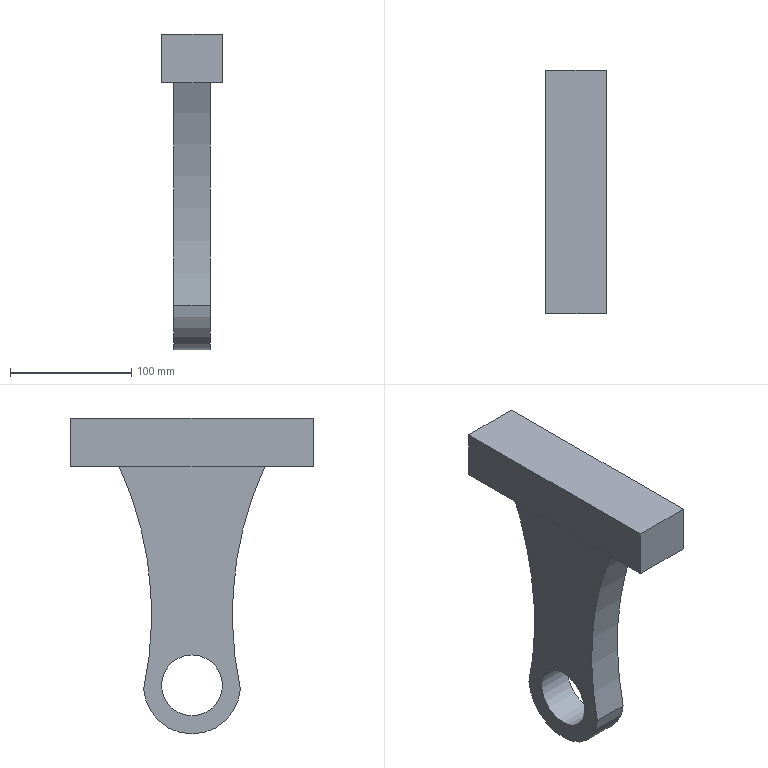Component | NX | HAMMER_HEAD_3 | 1 solid | 12 faces | box 50 x 200 x 260 mm | volume 846348 mm3 | plane 8 | cylinder 4 | commonest cylinder face diameters 580.798 x2 80 x1 50 x1
STEP:
#1=CARTESIAN_POINT('',(0.,0.,0.));
#2=DIRECTION('',(0.,0.,1.));
#3=DIRECTION('',(1.,0.,0.));
#4=AXIS2_PLACEMENT_3D('',#1,#2,#3);
#5=CARTESIAN_POINT('',(660.371,-609.017,1839.037));
#6=VERTEX_POINT('',#5);
#7=CARTESIAN_POINT('',(660.371,-688.747,1839.037));
#8=VERTEX_POINT('',#7);
#9=CARTESIAN_POINT('',(660.371,-648.882,1842.318));
#10=DIRECTION('',(-1.,0.,0.));
#11=DIRECTION('',(0.,0.,1.));
#12=AXIS2_PLACEMENT_3D('',#9,#10,#11);
#13=CIRCLE('',#12,40.);
#14=CARTESIAN_POINT('',(630.371,-648.882,1842.318));
#15=DIRECTION('',(1.,0.,0.));
#16=DIRECTION('',(0.,0.,-1.));
#17=AXIS2_PLACEMENT_3D('',#14,#15,#16);
#18=CYLINDRICAL_SURFACE('',#17,40.);
#19=CARTESIAN_POINT('',(3.142,30.));
#20=DIRECTION('',(-1.,0.));
#21=VECTOR('',#20,1.);
#22=LINE('',#19,#21);
#23=(GEOMETRIC_REPRESENTATION_CONTEXT(2)PARAMETRIC_REPRESENTATION_CONTEXT()REPRESENTATION_CONTEXT('',''));
#24=DEFINITIONAL_REPRESENTATION('',(#22),#23);
#25=PCURVE('',#18,#24);
#26=CARTESIAN_POINT('',(660.371,-648.882,1842.318));
#27=DIRECTION('',(-1.,0.,0.));
#28=DIRECTION('',(0.,0.,1.));
#29=AXIS2_PLACEMENT_3D('',#26,#27,#28);
#30=PLANE('',#29);
#31=CARTESIAN_POINT('',(0.,0.));
#32=DIRECTION('',(1.,0.));
#33=AXIS2_PLACEMENT_2D('',#31,#32);
#34=CIRCLE('',#33,40.);
#35=(GEOMETRIC_REPRESENTATION_CONTEXT(2)PARAMETRIC_REPRESENTATION_CONTEXT()REPRESENTATION_CONTEXT('',''));
#36=DEFINITIONAL_REPRESENTATION('',(#34),#35);
#37=PCURVE('',#30,#36);
#38=SURFACE_CURVE('',#13,(#25,#37),.PCURVE_S1.);
#39=EDGE_CURVE('',#6,#8,#38,.T.);
#40=ORIENTED_EDGE('',*,*,#39,.T.);
#41=CARTESIAN_POINT('',(630.371,-688.747,1839.037));
#42=VERTEX_POINT('',#41);
#43=CARTESIAN_POINT('',(630.371,-688.747,1839.037));
#44=DIRECTION('',(1.,0.,0.));
#45=VECTOR('',#44,1.);
#46=LINE('',#43,#45);
#47=CARTESIAN_POINT('',(-1.489,0.));
#48=DIRECTION('',(0.,1.));
#49=VECTOR('',#48,1.);
#50=LINE('',#47,#49);
#51=(GEOMETRIC_REPRESENTATION_CONTEXT(2)PARAMETRIC_REPRESENTATION_CONTEXT()REPRESENTATION_CONTEXT('',''));
#52=DEFINITIONAL_REPRESENTATION('',(#50),#51);
#53=PCURVE('',#18,#52);
#54=CARTESIAN_POINT('',(630.371,-972.544,1900.606));
#55=DIRECTION('',(1.,0.,0.));
#56=DIRECTION('',(0.,0.,-1.));
#57=AXIS2_PLACEMENT_3D('',#54,#55,#56);
#58=CYLINDRICAL_SURFACE('',#57,290.399);
#59=CARTESIAN_POINT('',(1.357,0.));
#60=DIRECTION('',(0.,1.));
#61=VECTOR('',#60,1.);
#62=LINE('',#59,#61);
#63=(GEOMETRIC_REPRESENTATION_CONTEXT(2)PARAMETRIC_REPRESENTATION_CONTEXT()REPRESENTATION_CONTEXT('',''));
#64=DEFINITIONAL_REPRESENTATION('',(#62),#63);
#65=PCURVE('',#58,#64);
#66=SURFACE_CURVE('',#46,(#53,#65),.PCURVE_S1.);
#67=EDGE_CURVE('',#42,#8,#66,.T.);
#68=ORIENTED_EDGE('',*,*,#67,.F.);
#69=CARTESIAN_POINT('',(630.371,-609.017,1839.037));
#70=VERTEX_POINT('',#69);
#71=CARTESIAN_POINT('',(630.371,-648.882,1842.318));
#72=DIRECTION('',(-1.,0.,0.));
#73=DIRECTION('',(0.,0.,1.));
#74=AXIS2_PLACEMENT_3D('',#71,#72,#73);
#75=CIRCLE('',#74,40.);
#76=CARTESIAN_POINT('',(3.142,0.));
#77=DIRECTION('',(-1.,0.));
#78=VECTOR('',#77,1.);
#79=LINE('',#76,#78);
#80=(GEOMETRIC_REPRESENTATION_CONTEXT(2)PARAMETRIC_REPRESENTATION_CONTEXT()REPRESENTATION_CONTEXT('',''));
#81=DEFINITIONAL_REPRESENTATION('',(#79),#80);
#82=PCURVE('',#18,#81);
#83=CARTESIAN_POINT('',(630.371,-648.882,1842.318));
#84=DIRECTION('',(-1.,0.,0.));
#85=DIRECTION('',(0.,0.,1.));
#86=AXIS2_PLACEMENT_3D('',#83,#84,#85);
#87=PLANE('',#86);
#88=CARTESIAN_POINT('',(0.,0.));
#89=DIRECTION('',(1.,0.));
#90=AXIS2_PLACEMENT_2D('',#88,#89);
#91=CIRCLE('',#90,40.);
#92=(GEOMETRIC_REPRESENTATION_CONTEXT(2)PARAMETRIC_REPRESENTATION_CONTEXT()REPRESENTATION_CONTEXT('',''));
#93=DEFINITIONAL_REPRESENTATION('',(#91),#92);
#94=PCURVE('',#87,#93);
#95=SURFACE_CURVE('',#75,(#82,#94),.PCURVE_S1.);
#96=EDGE_CURVE('',#70,#42,#95,.T.);
#97=ORIENTED_EDGE('',*,*,#96,.F.);
#98=CARTESIAN_POINT('',(630.371,-609.017,1839.037));
#99=DIRECTION('',(1.,0.,0.));
#100=VECTOR('',#99,1.);
#101=LINE('',#98,#100);
#102=CARTESIAN_POINT('',(1.489,0.));
#103=DIRECTION('',(0.,1.));
#104=VECTOR('',#103,1.);
#105=LINE('',#102,#104);
#106=(GEOMETRIC_REPRESENTATION_CONTEXT(2)PARAMETRIC_REPRESENTATION_CONTEXT()REPRESENTATION_CONTEXT('',''));
#107=DEFINITIONAL_REPRESENTATION('',(#105),#106);
#108=PCURVE('',#18,#107);
#109=CARTESIAN_POINT('',(630.371,-325.22,1900.606));
#110=DIRECTION('',(1.,0.,0.));
#111=DIRECTION('',(0.,0.,-1.));
#112=AXIS2_PLACEMENT_3D('',#109,#110,#111);
#113=CYLINDRICAL_SURFACE('',#112,290.399);
#114=CARTESIAN_POINT('',(4.926,0.));
#115=DIRECTION('',(0.,1.));
#116=VECTOR('',#115,1.);
#117=LINE('',#114,#116);
#118=(GEOMETRIC_REPRESENTATION_CONTEXT(2)PARAMETRIC_REPRESENTATION_CONTEXT()REPRESENTATION_CONTEXT('',''));
#119=DEFINITIONAL_REPRESENTATION('',(#117),#118);
#120=PCURVE('',#113,#119);
#121=SURFACE_CURVE('',#101,(#108,#120),.PCURVE_S1.);
#122=EDGE_CURVE('',#70,#6,#121,.T.);
#123=ORIENTED_EDGE('',*,*,#122,.T.);
#124=EDGE_LOOP('',(#40,#68,#97,#123));
#125=FACE_BOUND('',#124,.T.);
#126=ADVANCED_FACE('',(#125),#18,.T.);
#127=ORIENTED_EDGE('',*,*,#67,.F.);
#128=CARTESIAN_POINT('',(630.371,-708.882,2022.318));
#129=VERTEX_POINT('',#128);
#130=CARTESIAN_POINT('',(630.371,-972.544,1900.606));
#131=DIRECTION('',(1.,0.,0.));
#132=DIRECTION('',(0.,0.,1.));
#133=AXIS2_PLACEMENT_3D('',#130,#131,#132);
#134=CIRCLE('',#133,290.399);
#135=CARTESIAN_POINT('',(-3.142,0.));
#136=DIRECTION('',(1.,0.));
#137=VECTOR('',#136,1.);
#138=LINE('',#135,#137);
#139=(GEOMETRIC_REPRESENTATION_CONTEXT(2)PARAMETRIC_REPRESENTATION_CONTEXT()REPRESENTATION_CONTEXT('',''));
#140=DEFINITIONAL_REPRESENTATION('',(#138),#139);
#141=PCURVE('',#58,#140);
#142=CARTESIAN_POINT('',(348.687,-323.662));
#143=CARTESIAN_POINT('',(348.687,-826.648));
#144=CARTESIAN_POINT('',(-86.911,-575.155));
#145=CARTESIAN_POINT('',(-522.509,-323.662));
#146=CARTESIAN_POINT('',(-86.911,-72.169));
#147=CARTESIAN_POINT('',(348.687,179.323));
#148=CARTESIAN_POINT('',(348.687,-323.662));
#149=(BOUNDED_CURVE()B_SPLINE_CURVE(2,(#142,#143,#144,#145,#146,#147,#148),.UNSPECIFIED.,.T.,.F.)B_SPLINE_CURVE_WITH_KNOTS((1,2,2,2,2,1),(-2.094,0.,2.094,4.189,6.283,8.378),.UNSPECIFIED.)CURVE()GEOMETRIC_REPRESENTATION_ITEM()RATIONAL_B_SPLINE_CURVE((1.,0.5,1.,0.5,1.,0.5,1.))REPRESENTATION_ITEM(''));
#150=(GEOMETRIC_REPRESENTATION_CONTEXT(2)PARAMETRIC_REPRESENTATION_CONTEXT()REPRESENTATION_CONTEXT('',''));
#151=DEFINITIONAL_REPRESENTATION('',(#149),#150);
#152=PCURVE('',#87,#151);
#153=SURFACE_CURVE('',#134,(#141,#152),.PCURVE_S1.);
#154=EDGE_CURVE('',#42,#129,#153,.T.);
#155=ORIENTED_EDGE('',*,*,#154,.T.);
#156=CARTESIAN_POINT('',(660.371,-708.882,2022.318));
#157=VERTEX_POINT('',#156);
#158=CARTESIAN_POINT('',(630.371,-708.882,2022.318));
#159=DIRECTION('',(1.,0.,0.));
#160=VECTOR('',#159,1.);
#161=LINE('',#158,#160);
#162=CARTESIAN_POINT('',(2.003,0.));
#163=DIRECTION('',(0.,1.));
#164=VECTOR('',#163,1.);
#165=LINE('',#162,#164);
#166=(GEOMETRIC_REPRESENTATION_CONTEXT(2)PARAMETRIC_REPRESENTATION_CONTEXT()REPRESENTATION_CONTEXT('',''));
#167=DEFINITIONAL_REPRESENTATION('',(#165),#166);
#168=PCURVE('',#58,#167);
#169=CARTESIAN_POINT('',(660.371,-648.882,2022.318));
#170=DIRECTION('',(0.,-0.,1.));
#171=DIRECTION('',(0.,1.,0.));
#172=AXIS2_PLACEMENT_3D('',#169,#170,#171);
#173=PLANE('',#172);
#174=CARTESIAN_POINT('',(-60.,30.));
#175=DIRECTION('',(0.,-1.));
#176=VECTOR('',#175,1.);
#177=LINE('',#174,#176);
#178=(GEOMETRIC_REPRESENTATION_CONTEXT(2)PARAMETRIC_REPRESENTATION_CONTEXT()REPRESENTATION_CONTEXT('',''));
#179=DEFINITIONAL_REPRESENTATION('',(#177),#178);
#180=PCURVE('',#173,#179);
#181=SURFACE_CURVE('',#161,(#168,#180),.PCURVE_S1.);
#182=EDGE_CURVE('',#129,#157,#181,.T.);
#183=ORIENTED_EDGE('',*,*,#182,.T.);
#184=CARTESIAN_POINT('',(660.371,-972.544,1900.606));
#185=DIRECTION('',(1.,0.,0.));
#186=DIRECTION('',(0.,0.,1.));
#187=AXIS2_PLACEMENT_3D('',#184,#185,#186);
#188=CIRCLE('',#187,290.399);
#189=CARTESIAN_POINT('',(-3.142,30.));
#190=DIRECTION('',(1.,0.));
#191=VECTOR('',#190,1.);
#192=LINE('',#189,#191);
#193=(GEOMETRIC_REPRESENTATION_CONTEXT(2)PARAMETRIC_REPRESENTATION_CONTEXT()REPRESENTATION_CONTEXT('',''));
#194=DEFINITIONAL_REPRESENTATION('',(#192),#193);
#195=PCURVE('',#58,#194);
#196=CARTESIAN_POINT('',(348.687,-323.662));
#197=CARTESIAN_POINT('',(348.687,-826.648));
#198=CARTESIAN_POINT('',(-86.911,-575.155));
#199=CARTESIAN_POINT('',(-522.509,-323.662));
#200=CARTESIAN_POINT('',(-86.911,-72.169));
#201=CARTESIAN_POINT('',(348.687,179.323));
#202=CARTESIAN_POINT('',(348.687,-323.662));
#203=(BOUNDED_CURVE()B_SPLINE_CURVE(2,(#196,#197,#198,#199,#200,#201,#202),.UNSPECIFIED.,.T.,.F.)B_SPLINE_CURVE_WITH_KNOTS((1,2,2,2,2,1),(-2.094,0.,2.094,4.189,6.283,8.378),.UNSPECIFIED.)CURVE()GEOMETRIC_REPRESENTATION_ITEM()RATIONAL_B_SPLINE_CURVE((1.,0.5,1.,0.5,1.,0.5,1.))REPRESENTATION_ITEM(''));
#204=(GEOMETRIC_REPRESENTATION_CONTEXT(2)PARAMETRIC_REPRESENTATION_CONTEXT()REPRESENTATION_CONTEXT('',''));
#205=DEFINITIONAL_REPRESENTATION('',(#203),#204);
#206=PCURVE('',#30,#205);
#207=SURFACE_CURVE('',#188,(#195,#206),.PCURVE_S1.);
#208=EDGE_CURVE('',#8,#157,#207,.T.);
#209=ORIENTED_EDGE('',*,*,#208,.F.);
#210=EDGE_LOOP('',(#127,#155,#183,#209));
#211=FACE_BOUND('',#210,.F.);
#212=ADVANCED_FACE('',(#211),#58,.F.);
#213=CARTESIAN_POINT('',(630.371,-588.882,2022.318));
#214=VERTEX_POINT('',#213);
#215=CARTESIAN_POINT('',(660.371,-588.882,2022.318));
#216=VERTEX_POINT('',#215);
#217=CARTESIAN_POINT('',(630.371,-588.882,2022.318));
#218=DIRECTION('',(1.,0.,0.));
#219=VECTOR('',#218,1.);
#220=LINE('',#217,#219);
#221=CARTESIAN_POINT('',(4.28,0.));
#222=DIRECTION('',(0.,1.));
#223=VECTOR('',#222,1.);
#224=LINE('',#221,#223);
#225=(GEOMETRIC_REPRESENTATION_CONTEXT(2)PARAMETRIC_REPRESENTATION_CONTEXT()REPRESENTATION_CONTEXT('',''));
#226=DEFINITIONAL_REPRESENTATION('',(#224),#225);
#227=PCURVE('',#113,#226);
#228=CARTESIAN_POINT('',(60.,30.));
#229=DIRECTION('',(0.,-1.));
#230=VECTOR('',#229,1.);
#231=LINE('',#228,#230);
#232=(GEOMETRIC_REPRESENTATION_CONTEXT(2)PARAMETRIC_REPRESENTATION_CONTEXT()REPRESENTATION_CONTEXT('',''));
#233=DEFINITIONAL_REPRESENTATION('',(#231),#232);
#234=PCURVE('',#173,#233);
#235=SURFACE_CURVE('',#220,(#227,#234),.PCURVE_S1.);
#236=EDGE_CURVE('',#214,#216,#235,.T.);
#237=ORIENTED_EDGE('',*,*,#236,.F.);
#238=CARTESIAN_POINT('',(630.371,-325.22,1900.606));
#239=DIRECTION('',(1.,0.,0.));
#240=DIRECTION('',(0.,0.,1.));
#241=AXIS2_PLACEMENT_3D('',#238,#239,#240);
#242=CIRCLE('',#241,290.399);
#243=CARTESIAN_POINT('',(3.142,0.));
#244=DIRECTION('',(1.,0.));
#245=VECTOR('',#244,1.);
#246=LINE('',#243,#245);
#247=(GEOMETRIC_REPRESENTATION_CONTEXT(2)PARAMETRIC_REPRESENTATION_CONTEXT()REPRESENTATION_CONTEXT('',''));
#248=DEFINITIONAL_REPRESENTATION('',(#246),#247);
#249=PCURVE('',#113,#248);
#250=CARTESIAN_POINT('',(348.687,323.662));
#251=CARTESIAN_POINT('',(348.687,-179.323));
#252=CARTESIAN_POINT('',(-86.911,72.169));
#253=CARTESIAN_POINT('',(-522.509,323.662));
#254=CARTESIAN_POINT('',(-86.911,575.155));
#255=CARTESIAN_POINT('',(348.687,826.648));
#256=CARTESIAN_POINT('',(348.687,323.662));
#257=(BOUNDED_CURVE()B_SPLINE_CURVE(2,(#250,#251,#252,#253,#254,#255,#256),.UNSPECIFIED.,.T.,.F.)B_SPLINE_CURVE_WITH_KNOTS((1,2,2,2,2,1),(-2.094,0.,2.094,4.189,6.283,8.378),.UNSPECIFIED.)CURVE()GEOMETRIC_REPRESENTATION_ITEM()RATIONAL_B_SPLINE_CURVE((1.,0.5,1.,0.5,1.,0.5,1.))REPRESENTATION_ITEM(''));
#258=(GEOMETRIC_REPRESENTATION_CONTEXT(2)PARAMETRIC_REPRESENTATION_CONTEXT()REPRESENTATION_CONTEXT('',''));
#259=DEFINITIONAL_REPRESENTATION('',(#257),#258);
#260=PCURVE('',#87,#259);
#261=SURFACE_CURVE('',#242,(#249,#260),.PCURVE_S1.);
#262=EDGE_CURVE('',#214,#70,#261,.T.);
#263=ORIENTED_EDGE('',*,*,#262,.T.);
#264=ORIENTED_EDGE('',*,*,#122,.T.);
#265=CARTESIAN_POINT('',(660.371,-325.22,1900.606));
#266=DIRECTION('',(1.,0.,0.));
#267=DIRECTION('',(0.,0.,1.));
#268=AXIS2_PLACEMENT_3D('',#265,#266,#267);
#269=CIRCLE('',#268,290.399);
#270=CARTESIAN_POINT('',(3.142,30.));
#271=DIRECTION('',(1.,0.));
#272=VECTOR('',#271,1.);
#273=LINE('',#270,#272);
#274=(GEOMETRIC_REPRESENTATION_CONTEXT(2)PARAMETRIC_REPRESENTATION_CONTEXT()REPRESENTATION_CONTEXT('',''));
#275=DEFINITIONAL_REPRESENTATION('',(#273),#274);
#276=PCURVE('',#113,#275);
#277=CARTESIAN_POINT('',(348.687,323.662));
#278=CARTESIAN_POINT('',(348.687,-179.323));
#279=CARTESIAN_POINT('',(-86.911,72.169));
#280=CARTESIAN_POINT('',(-522.509,323.662));
#281=CARTESIAN_POINT('',(-86.911,575.155));
#282=CARTESIAN_POINT('',(348.687,826.648));
#283=CARTESIAN_POINT('',(348.687,323.662));
#284=(BOUNDED_CURVE()B_SPLINE_CURVE(2,(#277,#278,#279,#280,#281,#282,#283),.UNSPECIFIED.,.T.,.F.)B_SPLINE_CURVE_WITH_KNOTS((1,2,2,2,2,1),(-2.094,0.,2.094,4.189,6.283,8.378),.UNSPECIFIED.)CURVE()GEOMETRIC_REPRESENTATION_ITEM()RATIONAL_B_SPLINE_CURVE((1.,0.5,1.,0.5,1.,0.5,1.))REPRESENTATION_ITEM(''));
#285=(GEOMETRIC_REPRESENTATION_CONTEXT(2)PARAMETRIC_REPRESENTATION_CONTEXT()REPRESENTATION_CONTEXT('',''));
#286=DEFINITIONAL_REPRESENTATION('',(#284),#285);
#287=PCURVE('',#30,#286);
#288=SURFACE_CURVE('',#269,(#276,#287),.PCURVE_S1.);
#289=EDGE_CURVE('',#216,#6,#288,.T.);
#290=ORIENTED_EDGE('',*,*,#289,.F.);
#291=EDGE_LOOP('',(#237,#263,#264,#290));
#292=FACE_BOUND('',#291,.F.);
#293=ADVANCED_FACE('',(#292),#113,.F.);
#294=CARTESIAN_POINT('',(630.371,-648.882,1867.318));
#295=VERTEX_POINT('',#294);
#296=CARTESIAN_POINT('',(630.371,-648.882,1842.318));
#297=DIRECTION('',(-1.,0.,0.));
#298=DIRECTION('',(0.,0.,1.));
#299=AXIS2_PLACEMENT_3D('',#296,#297,#298);
#300=CIRCLE('',#299,25.);
#301=CARTESIAN_POINT('',(630.371,-648.882,1842.318));
#302=DIRECTION('',(1.,0.,0.));
#303=DIRECTION('',(0.,0.,-1.));
#304=AXIS2_PLACEMENT_3D('',#301,#302,#303);
#305=CYLINDRICAL_SURFACE('',#304,25.);
#306=CARTESIAN_POINT('',(9.425,0.));
#307=DIRECTION('',(-1.,0.));
#308=VECTOR('',#307,1.);
#309=LINE('',#306,#308);
#310=(GEOMETRIC_REPRESENTATION_CONTEXT(2)PARAMETRIC_REPRESENTATION_CONTEXT()REPRESENTATION_CONTEXT('',''));
#311=DEFINITIONAL_REPRESENTATION('',(#309),#310);
#312=PCURVE('',#305,#311);
#313=CARTESIAN_POINT('',(0.,0.));
#314=DIRECTION('',(1.,0.));
#315=AXIS2_PLACEMENT_2D('',#313,#314);
#316=CIRCLE('',#315,25.);
#317=(GEOMETRIC_REPRESENTATION_CONTEXT(2)PARAMETRIC_REPRESENTATION_CONTEXT()REPRESENTATION_CONTEXT('',''));
#318=DEFINITIONAL_REPRESENTATION('',(#316),#317);
#319=PCURVE('',#87,#318);
#320=SURFACE_CURVE('',#300,(#312,#319),.PCURVE_S1.);
#321=EDGE_CURVE('',#295,#295,#320,.T.);
#322=ORIENTED_EDGE('',*,*,#321,.F.);
#323=CARTESIAN_POINT('',(660.371,-648.882,1867.318));
#324=VERTEX_POINT('',#323);
#325=CARTESIAN_POINT('',(630.371,-648.882,1867.318));
#326=CARTESIAN_POINT('',(660.371,-648.882,1867.318));
#327=B_SPLINE_CURVE_WITH_KNOTS('',1,(#325,#326),.UNSPECIFIED.,.F.,.F.,(2,2),(0.,30.),.PIECEWISE_BEZIER_KNOTS.);
#328=CARTESIAN_POINT('',(9.425,0.));
#329=DIRECTION('',(0.,1.));
#330=VECTOR('',#329,1.);
#331=LINE('',#328,#330);
#332=(GEOMETRIC_REPRESENTATION_CONTEXT(2)PARAMETRIC_REPRESENTATION_CONTEXT()REPRESENTATION_CONTEXT('',''));
#333=DEFINITIONAL_REPRESENTATION('',(#331),#332);
#334=PCURVE('',#305,#333);
#335=CARTESIAN_POINT('',(3.142,0.));
#336=DIRECTION('',(0.,1.));
#337=VECTOR('',#336,1.);
#338=LINE('',#335,#337);
#339=(GEOMETRIC_REPRESENTATION_CONTEXT(2)PARAMETRIC_REPRESENTATION_CONTEXT()REPRESENTATION_CONTEXT('',''));
#340=DEFINITIONAL_REPRESENTATION('',(#338),#339);
#341=PCURVE('',#305,#340);
#342=SEAM_CURVE('',#327,(#334,#341),.PCURVE_S1.);
#343=EDGE_CURVE('',#295,#324,#342,.T.);
#344=ORIENTED_EDGE('',*,*,#343,.T.);
#345=CARTESIAN_POINT('',(660.371,-648.882,1842.318));
#346=DIRECTION('',(-1.,0.,0.));
#347=DIRECTION('',(0.,0.,1.));
#348=AXIS2_PLACEMENT_3D('',#345,#346,#347);
#349=CIRCLE('',#348,25.);
#350=CARTESIAN_POINT('',(9.425,30.));
#351=DIRECTION('',(-1.,0.));
#352=VECTOR('',#351,1.);
#353=LINE('',#350,#352);
#354=(GEOMETRIC_REPRESENTATION_CONTEXT(2)PARAMETRIC_REPRESENTATION_CONTEXT()REPRESENTATION_CONTEXT('',''));
#355=DEFINITIONAL_REPRESENTATION('',(#353),#354);
#356=PCURVE('',#305,#355);
#357=CARTESIAN_POINT('',(0.,0.));
#358=DIRECTION('',(1.,0.));
#359=AXIS2_PLACEMENT_2D('',#357,#358);
#360=CIRCLE('',#359,25.);
#361=(GEOMETRIC_REPRESENTATION_CONTEXT(2)PARAMETRIC_REPRESENTATION_CONTEXT()REPRESENTATION_CONTEXT('',''));
#362=DEFINITIONAL_REPRESENTATION('',(#360),#361);
#363=PCURVE('',#30,#362);
#364=SURFACE_CURVE('',#349,(#356,#363),.PCURVE_S1.);
#365=EDGE_CURVE('',#324,#324,#364,.T.);
#366=ORIENTED_EDGE('',*,*,#365,.T.);
#367=ORIENTED_EDGE('',*,*,#343,.F.);
#368=EDGE_LOOP('',(#322,#344,#366,#367));
#369=FACE_BOUND('',#368,.F.);
#370=ADVANCED_FACE('',(#369),#305,.F.);
#371=ORIENTED_EDGE('',*,*,#96,.T.);
#372=ORIENTED_EDGE('',*,*,#154,.T.);
#373=CARTESIAN_POINT('',(630.371,-708.882,2022.318));
#374=DIRECTION('',(0.,1.,0.));
#375=VECTOR('',#374,1.);
#376=LINE('',#373,#375);
#377=CARTESIAN_POINT('',(180.,-60.));
#378=DIRECTION('',(0.,1.));
#379=VECTOR('',#378,1.);
#380=LINE('',#377,#379);
#381=(GEOMETRIC_REPRESENTATION_CONTEXT(2)PARAMETRIC_REPRESENTATION_CONTEXT()REPRESENTATION_CONTEXT('',''));
#382=DEFINITIONAL_REPRESENTATION('',(#380),#381);
#383=PCURVE('',#87,#382);
#384=CARTESIAN_POINT('',(-60.,30.));
#385=DIRECTION('',(1.,0.));
#386=VECTOR('',#385,1.);
#387=LINE('',#384,#386);
#388=(GEOMETRIC_REPRESENTATION_CONTEXT(2)PARAMETRIC_REPRESENTATION_CONTEXT()REPRESENTATION_CONTEXT('',''));
#389=DEFINITIONAL_REPRESENTATION('',(#387),#388);
#390=PCURVE('',#173,#389);
#391=SURFACE_CURVE('',#376,(#383,#390),.PCURVE_S1.);
#392=EDGE_CURVE('',#129,#214,#391,.T.);
#393=ORIENTED_EDGE('',*,*,#392,.T.);
#394=ORIENTED_EDGE('',*,*,#262,.T.);
#395=EDGE_LOOP('',(#371,#372,#393,#394));
#396=FACE_BOUND('',#395,.T.);
#397=ORIENTED_EDGE('',*,*,#321,.F.);
#398=EDGE_LOOP('',(#397));
#399=FACE_BOUND('',#398,.T.);
#400=ADVANCED_FACE('',(#396,#399),#87,.T.);
#401=ORIENTED_EDGE('',*,*,#39,.F.);
#402=ORIENTED_EDGE('',*,*,#289,.F.);
#403=CARTESIAN_POINT('',(660.371,-648.882,2022.318));
#404=DIRECTION('',(0.,1.,0.));
#405=VECTOR('',#404,1.);
#406=LINE('',#403,#405);
#407=CARTESIAN_POINT('',(180.,0.));
#408=DIRECTION('',(0.,1.));
#409=VECTOR('',#408,1.);
#410=LINE('',#407,#409);
#411=(GEOMETRIC_REPRESENTATION_CONTEXT(2)PARAMETRIC_REPRESENTATION_CONTEXT()REPRESENTATION_CONTEXT('',''));
#412=DEFINITIONAL_REPRESENTATION('',(#410),#411);
#413=PCURVE('',#30,#412);
#414=CARTESIAN_POINT('',(0.,0.));
#415=DIRECTION('',(1.,0.));
#416=VECTOR('',#415,1.);
#417=LINE('',#414,#416);
#418=(GEOMETRIC_REPRESENTATION_CONTEXT(2)PARAMETRIC_REPRESENTATION_CONTEXT()REPRESENTATION_CONTEXT('',''));
#419=DEFINITIONAL_REPRESENTATION('',(#417),#418);
#420=PCURVE('',#173,#419);
#421=SURFACE_CURVE('',#406,(#413,#420),.PCURVE_S1.);
#422=EDGE_CURVE('',#157,#216,#421,.T.);
#423=ORIENTED_EDGE('',*,*,#422,.F.);
#424=ORIENTED_EDGE('',*,*,#208,.F.);
#425=EDGE_LOOP('',(#401,#402,#423,#424));
#426=FACE_BOUND('',#425,.T.);
#427=ORIENTED_EDGE('',*,*,#365,.T.);
#428=EDGE_LOOP('',(#427));
#429=FACE_BOUND('',#428,.T.);
#430=ADVANCED_FACE('',(#426,#429),#30,.F.);
#431=CARTESIAN_POINT('',(620.371,-748.882,2022.318));
#432=VERTEX_POINT('',#431);
#433=CARTESIAN_POINT('',(670.371,-748.882,2022.318));
#434=VERTEX_POINT('',#433);
#435=CARTESIAN_POINT('',(620.371,-748.882,2022.318));
#436=DIRECTION('',(1.,0.,0.));
#437=VECTOR('',#436,1.);
#438=LINE('',#435,#437);
#439=CARTESIAN_POINT('',(-100.,40.));
#440=DIRECTION('',(0.,-1.));
#441=VECTOR('',#440,1.);
#442=LINE('',#439,#441);
#443=(GEOMETRIC_REPRESENTATION_CONTEXT(2)PARAMETRIC_REPRESENTATION_CONTEXT()REPRESENTATION_CONTEXT('',''));
#444=DEFINITIONAL_REPRESENTATION('',(#442),#443);
#445=PCURVE('',#173,#444);
#446=CARTESIAN_POINT('',(620.371,-748.882,2062.318));
#447=DIRECTION('',(0.,1.,0.));
#448=DIRECTION('',(0.,0.,-1.));
#449=AXIS2_PLACEMENT_3D('',#446,#447,#448);
#450=PLANE('',#449);
#451=CARTESIAN_POINT('',(40.,0.));
#452=DIRECTION('',(0.,-1.));
#453=VECTOR('',#452,1.);
#454=LINE('',#451,#453);
#455=(GEOMETRIC_REPRESENTATION_CONTEXT(2)PARAMETRIC_REPRESENTATION_CONTEXT()REPRESENTATION_CONTEXT('',''));
#456=DEFINITIONAL_REPRESENTATION('',(#454),#455);
#457=PCURVE('',#450,#456);
#458=SURFACE_CURVE('',#438,(#445,#457),.PCURVE_S1.);
#459=EDGE_CURVE('',#432,#434,#458,.T.);
#460=ORIENTED_EDGE('',*,*,#459,.F.);
#461=CARTESIAN_POINT('',(620.371,-548.882,2022.318));
#462=VERTEX_POINT('',#461);
#463=CARTESIAN_POINT('',(620.371,-548.882,2022.318));
#464=DIRECTION('',(-0.,-1.,-0.));
#465=VECTOR('',#464,1.);
#466=LINE('',#463,#465);
#467=CARTESIAN_POINT('',(100.,40.));
#468=DIRECTION('',(-1.,0.));
#469=VECTOR('',#468,1.);
#470=LINE('',#467,#469);
#471=(GEOMETRIC_REPRESENTATION_CONTEXT(2)PARAMETRIC_REPRESENTATION_CONTEXT()REPRESENTATION_CONTEXT('',''));
#472=DEFINITIONAL_REPRESENTATION('',(#470),#471);
#473=PCURVE('',#173,#472);
#474=CARTESIAN_POINT('',(620.371,-548.882,2062.318));
#475=DIRECTION('',(1.,-0.,-0.));
#476=DIRECTION('',(0.,1.,-0.));
#477=AXIS2_PLACEMENT_3D('',#474,#475,#476);
#478=PLANE('',#477);
#479=CARTESIAN_POINT('',(0.,-40.));
#480=DIRECTION('',(-1.,-0.));
#481=VECTOR('',#480,1.);
#482=LINE('',#479,#481);
#483=(GEOMETRIC_REPRESENTATION_CONTEXT(2)PARAMETRIC_REPRESENTATION_CONTEXT()REPRESENTATION_CONTEXT('',''));
#484=DEFINITIONAL_REPRESENTATION('',(#482),#483);
#485=PCURVE('',#478,#484);
#486=SURFACE_CURVE('',#466,(#473,#485),.PCURVE_S1.);
#487=EDGE_CURVE('',#462,#432,#486,.T.);
#488=ORIENTED_EDGE('',*,*,#487,.F.);
#489=CARTESIAN_POINT('',(670.371,-548.882,2022.318));
#490=VERTEX_POINT('',#489);
#491=CARTESIAN_POINT('',(670.371,-548.882,2022.318));
#492=DIRECTION('',(-1.,0.,0.));
#493=VECTOR('',#492,1.);
#494=LINE('',#491,#493);
#495=CARTESIAN_POINT('',(100.,-10.));
#496=DIRECTION('',(0.,1.));
#497=VECTOR('',#496,1.);
#498=LINE('',#495,#497);
#499=(GEOMETRIC_REPRESENTATION_CONTEXT(2)PARAMETRIC_REPRESENTATION_CONTEXT()REPRESENTATION_CONTEXT('',''));
#500=DEFINITIONAL_REPRESENTATION('',(#498),#499);
#501=PCURVE('',#173,#500);
#502=CARTESIAN_POINT('',(670.371,-548.882,2062.318));
#503=DIRECTION('',(-0.,-1.,-0.));
#504=DIRECTION('',(1.,-0.,0.));
#505=AXIS2_PLACEMENT_3D('',#502,#503,#504);
#506=PLANE('',#505);
#507=CARTESIAN_POINT('',(0.,-40.));
#508=DIRECTION('',(-1.,0.));
#509=VECTOR('',#508,1.);
#510=LINE('',#507,#509);
#511=(GEOMETRIC_REPRESENTATION_CONTEXT(2)PARAMETRIC_REPRESENTATION_CONTEXT()REPRESENTATION_CONTEXT('',''));
#512=DEFINITIONAL_REPRESENTATION('',(#510),#511);
#513=PCURVE('',#506,#512);
#514=SURFACE_CURVE('',#494,(#501,#513),.PCURVE_S1.);
#515=EDGE_CURVE('',#490,#462,#514,.T.);
#516=ORIENTED_EDGE('',*,*,#515,.F.);
#517=CARTESIAN_POINT('',(670.371,-588.882,2022.318));
#518=DIRECTION('',(0.,1.,0.));
#519=VECTOR('',#518,1.);
#520=LINE('',#517,#519);
#521=CARTESIAN_POINT('',(60.,-10.));
#522=DIRECTION('',(1.,-0.));
#523=VECTOR('',#522,1.);
#524=LINE('',#521,#523);
#525=(GEOMETRIC_REPRESENTATION_CONTEXT(2)PARAMETRIC_REPRESENTATION_CONTEXT()REPRESENTATION_CONTEXT('',''));
#526=DEFINITIONAL_REPRESENTATION('',(#524),#525);
#527=PCURVE('',#173,#526);
#528=CARTESIAN_POINT('',(670.371,-588.882,2062.318));
#529=DIRECTION('',(-1.,0.,0.));
#530=DIRECTION('',(-0.,-1.,-0.));
#531=AXIS2_PLACEMENT_3D('',#528,#529,#530);
#532=PLANE('',#531);
#533=CARTESIAN_POINT('',(0.,-40.));
#534=DIRECTION('',(-1.,0.));
#535=VECTOR('',#534,1.);
#536=LINE('',#533,#535);
#537=(GEOMETRIC_REPRESENTATION_CONTEXT(2)PARAMETRIC_REPRESENTATION_CONTEXT()REPRESENTATION_CONTEXT('',''));
#538=DEFINITIONAL_REPRESENTATION('',(#536),#537);
#539=PCURVE('',#532,#538);
#540=SURFACE_CURVE('',#520,(#527,#539),.PCURVE_S1.);
#541=EDGE_CURVE('',#434,#490,#540,.T.);
#542=ORIENTED_EDGE('',*,*,#541,.F.);
#543=EDGE_LOOP('',(#460,#488,#516,#542));
#544=FACE_BOUND('',#543,.T.);
#545=ORIENTED_EDGE('',*,*,#182,.T.);
#546=ORIENTED_EDGE('',*,*,#422,.T.);
#547=ORIENTED_EDGE('',*,*,#236,.F.);
#548=ORIENTED_EDGE('',*,*,#392,.F.);
#549=EDGE_LOOP('',(#545,#546,#547,#548));
#550=FACE_BOUND('',#549,.T.);
#551=ADVANCED_FACE('',(#544,#550),#173,.F.);
#552=ORIENTED_EDGE('',*,*,#459,.T.);
#553=CARTESIAN_POINT('',(670.371,-748.882,2062.318));
#554=VERTEX_POINT('',#553);
#555=CARTESIAN_POINT('',(670.371,-748.882,2062.318));
#556=DIRECTION('',(0.,0.,-1.));
#557=VECTOR('',#556,1.);
#558=LINE('',#555,#557);
#559=CARTESIAN_POINT('',(0.,-50.));
#560=DIRECTION('',(1.,0.));
#561=VECTOR('',#560,1.);
#562=LINE('',#559,#561);
#563=(GEOMETRIC_REPRESENTATION_CONTEXT(2)PARAMETRIC_REPRESENTATION_CONTEXT()REPRESENTATION_CONTEXT('',''));
#564=DEFINITIONAL_REPRESENTATION('',(#562),#563);
#565=PCURVE('',#450,#564);
#566=CARTESIAN_POINT('',(160.,-0.));
#567=DIRECTION('',(-0.,-1.));
#568=VECTOR('',#567,1.);
#569=LINE('',#566,#568);
#570=(GEOMETRIC_REPRESENTATION_CONTEXT(2)PARAMETRIC_REPRESENTATION_CONTEXT()REPRESENTATION_CONTEXT('',''));
#571=DEFINITIONAL_REPRESENTATION('',(#569),#570);
#572=PCURVE('',#532,#571);
#573=SURFACE_CURVE('',#558,(#565,#572),.PCURVE_S1.);
#574=EDGE_CURVE('',#554,#434,#573,.T.);
#575=ORIENTED_EDGE('',*,*,#574,.F.);
#576=CARTESIAN_POINT('',(620.371,-748.882,2062.318));
#577=VERTEX_POINT('',#576);
#578=CARTESIAN_POINT('',(620.371,-748.882,2062.318));
#579=DIRECTION('',(1.,0.,0.));
#580=VECTOR('',#579,1.);
#581=LINE('',#578,#580);
#582=CARTESIAN_POINT('',(0.,0.));
#583=DIRECTION('',(0.,-1.));
#584=VECTOR('',#583,1.);
#585=LINE('',#582,#584);
#586=(GEOMETRIC_REPRESENTATION_CONTEXT(2)PARAMETRIC_REPRESENTATION_CONTEXT()REPRESENTATION_CONTEXT('',''));
#587=DEFINITIONAL_REPRESENTATION('',(#585),#586);
#588=PCURVE('',#450,#587);
#589=CARTESIAN_POINT('',(660.371,-648.882,2062.318));
#590=DIRECTION('',(0.,-0.,1.));
#591=DIRECTION('',(0.,1.,0.));
#592=AXIS2_PLACEMENT_3D('',#589,#590,#591);
#593=PLANE('',#592);
#594=CARTESIAN_POINT('',(-100.,40.));
#595=DIRECTION('',(0.,-1.));
#596=VECTOR('',#595,1.);
#597=LINE('',#594,#596);
#598=(GEOMETRIC_REPRESENTATION_CONTEXT(2)PARAMETRIC_REPRESENTATION_CONTEXT()REPRESENTATION_CONTEXT('',''));
#599=DEFINITIONAL_REPRESENTATION('',(#597),#598);
#600=PCURVE('',#593,#599);
#601=SURFACE_CURVE('',#581,(#588,#600),.PCURVE_S1.);
#602=EDGE_CURVE('',#577,#554,#601,.T.);
#603=ORIENTED_EDGE('',*,*,#602,.F.);
#604=CARTESIAN_POINT('',(620.371,-748.882,2062.318));
#605=DIRECTION('',(0.,0.,-1.));
#606=VECTOR('',#605,1.);
#607=LINE('',#604,#606);
#608=CARTESIAN_POINT('',(0.,0.));
#609=DIRECTION('',(1.,0.));
#610=VECTOR('',#609,1.);
#611=LINE('',#608,#610);
#612=(GEOMETRIC_REPRESENTATION_CONTEXT(2)PARAMETRIC_REPRESENTATION_CONTEXT()REPRESENTATION_CONTEXT('',''));
#613=DEFINITIONAL_REPRESENTATION('',(#611),#612);
#614=PCURVE('',#450,#613);
#615=CARTESIAN_POINT('',(-200.,-0.));
#616=DIRECTION('',(0.,-1.));
#617=VECTOR('',#616,1.);
#618=LINE('',#615,#617);
#619=(GEOMETRIC_REPRESENTATION_CONTEXT(2)PARAMETRIC_REPRESENTATION_CONTEXT()REPRESENTATION_CONTEXT('',''));
#620=DEFINITIONAL_REPRESENTATION('',(#618),#619);
#621=PCURVE('',#478,#620);
#622=SURFACE_CURVE('',#607,(#614,#621),.PCURVE_S1.);
#623=EDGE_CURVE('',#577,#432,#622,.T.);
#624=ORIENTED_EDGE('',*,*,#623,.T.);
#625=EDGE_LOOP('',(#552,#575,#603,#624));
#626=FACE_BOUND('',#625,.T.);
#627=ADVANCED_FACE('',(#626),#450,.F.);
#628=ORIENTED_EDGE('',*,*,#541,.T.);
#629=CARTESIAN_POINT('',(670.371,-548.882,2062.318));
#630=VERTEX_POINT('',#629);
#631=CARTESIAN_POINT('',(670.371,-548.882,2062.318));
#632=DIRECTION('',(0.,0.,-1.));
#633=VECTOR('',#632,1.);
#634=LINE('',#631,#633);
#635=CARTESIAN_POINT('',(-40.,-0.));
#636=DIRECTION('',(-0.,-1.));
#637=VECTOR('',#636,1.);
#638=LINE('',#635,#637);
#639=(GEOMETRIC_REPRESENTATION_CONTEXT(2)PARAMETRIC_REPRESENTATION_CONTEXT()REPRESENTATION_CONTEXT('',''));
#640=DEFINITIONAL_REPRESENTATION('',(#638),#639);
#641=PCURVE('',#532,#640);
#642=CARTESIAN_POINT('',(0.,0.));
#643=DIRECTION('',(-0.,-1.));
#644=VECTOR('',#643,1.);
#645=LINE('',#642,#644);
#646=(GEOMETRIC_REPRESENTATION_CONTEXT(2)PARAMETRIC_REPRESENTATION_CONTEXT()REPRESENTATION_CONTEXT('',''));
#647=DEFINITIONAL_REPRESENTATION('',(#645),#646);
#648=PCURVE('',#506,#647);
#649=SURFACE_CURVE('',#634,(#641,#648),.PCURVE_S1.);
#650=EDGE_CURVE('',#630,#490,#649,.T.);
#651=ORIENTED_EDGE('',*,*,#650,.F.);
#652=CARTESIAN_POINT('',(670.371,-748.882,2062.318));
#653=DIRECTION('',(0.,1.,0.));
#654=VECTOR('',#653,1.);
#655=LINE('',#652,#654);
#656=CARTESIAN_POINT('',(160.,-0.));
#657=DIRECTION('',(-1.,0.));
#658=VECTOR('',#657,1.);
#659=LINE('',#656,#658);
#660=(GEOMETRIC_REPRESENTATION_CONTEXT(2)PARAMETRIC_REPRESENTATION_CONTEXT()REPRESENTATION_CONTEXT('',''));
#661=DEFINITIONAL_REPRESENTATION('',(#659),#660);
#662=PCURVE('',#532,#661);
#663=CARTESIAN_POINT('',(-100.,-10.));
#664=DIRECTION('',(1.,-0.));
#665=VECTOR('',#664,1.);
#666=LINE('',#663,#665);
#667=(GEOMETRIC_REPRESENTATION_CONTEXT(2)PARAMETRIC_REPRESENTATION_CONTEXT()REPRESENTATION_CONTEXT('',''));
#668=DEFINITIONAL_REPRESENTATION('',(#666),#667);
#669=PCURVE('',#593,#668);
#670=SURFACE_CURVE('',#655,(#662,#669),.PCURVE_S1.);
#671=EDGE_CURVE('',#554,#630,#670,.T.);
#672=ORIENTED_EDGE('',*,*,#671,.F.);
#673=ORIENTED_EDGE('',*,*,#574,.T.);
#674=EDGE_LOOP('',(#628,#651,#672,#673));
#675=FACE_BOUND('',#674,.T.);
#676=ADVANCED_FACE('',(#675),#532,.F.);
#677=ORIENTED_EDGE('',*,*,#515,.T.);
#678=CARTESIAN_POINT('',(620.371,-548.882,2062.318));
#679=VERTEX_POINT('',#678);
#680=CARTESIAN_POINT('',(620.371,-548.882,2062.318));
#681=DIRECTION('',(0.,0.,-1.));
#682=VECTOR('',#681,1.);
#683=LINE('',#680,#682);
#684=CARTESIAN_POINT('',(-50.,-0.));
#685=DIRECTION('',(-0.,-1.));
#686=VECTOR('',#685,1.);
#687=LINE('',#684,#686);
#688=(GEOMETRIC_REPRESENTATION_CONTEXT(2)PARAMETRIC_REPRESENTATION_CONTEXT()REPRESENTATION_CONTEXT('',''));
#689=DEFINITIONAL_REPRESENTATION('',(#687),#688);
#690=PCURVE('',#506,#689);
#691=CARTESIAN_POINT('',(0.,0.));
#692=DIRECTION('',(0.,-1.));
#693=VECTOR('',#692,1.);
#694=LINE('',#691,#693);
#695=(GEOMETRIC_REPRESENTATION_CONTEXT(2)PARAMETRIC_REPRESENTATION_CONTEXT()REPRESENTATION_CONTEXT('',''));
#696=DEFINITIONAL_REPRESENTATION('',(#694),#695);
#697=PCURVE('',#478,#696);
#698=SURFACE_CURVE('',#683,(#690,#697),.PCURVE_S1.);
#699=EDGE_CURVE('',#679,#462,#698,.T.);
#700=ORIENTED_EDGE('',*,*,#699,.F.);
#701=CARTESIAN_POINT('',(670.371,-548.882,2062.318));
#702=DIRECTION('',(-1.,0.,0.));
#703=VECTOR('',#702,1.);
#704=LINE('',#701,#703);
#705=CARTESIAN_POINT('',(0.,0.));
#706=DIRECTION('',(-1.,0.));
#707=VECTOR('',#706,1.);
#708=LINE('',#705,#707);
#709=(GEOMETRIC_REPRESENTATION_CONTEXT(2)PARAMETRIC_REPRESENTATION_CONTEXT()REPRESENTATION_CONTEXT('',''));
#710=DEFINITIONAL_REPRESENTATION('',(#708),#709);
#711=PCURVE('',#506,#710);
#712=CARTESIAN_POINT('',(100.,-10.));
#713=DIRECTION('',(0.,1.));
#714=VECTOR('',#713,1.);
#715=LINE('',#712,#714);
#716=(GEOMETRIC_REPRESENTATION_CONTEXT(2)PARAMETRIC_REPRESENTATION_CONTEXT()REPRESENTATION_CONTEXT('',''));
#717=DEFINITIONAL_REPRESENTATION('',(#715),#716);
#718=PCURVE('',#593,#717);
#719=SURFACE_CURVE('',#704,(#711,#718),.PCURVE_S1.);
#720=EDGE_CURVE('',#630,#679,#719,.T.);
#721=ORIENTED_EDGE('',*,*,#720,.F.);
#722=ORIENTED_EDGE('',*,*,#650,.T.);
#723=EDGE_LOOP('',(#677,#700,#721,#722));
#724=FACE_BOUND('',#723,.T.);
#725=ADVANCED_FACE('',(#724),#506,.F.);
#726=ORIENTED_EDGE('',*,*,#487,.T.);
#727=ORIENTED_EDGE('',*,*,#623,.F.);
#728=CARTESIAN_POINT('',(620.371,-548.882,2062.318));
#729=DIRECTION('',(-0.,-1.,-0.));
#730=VECTOR('',#729,1.);
#731=LINE('',#728,#730);
#732=CARTESIAN_POINT('',(0.,0.));
#733=DIRECTION('',(-1.,-0.));
#734=VECTOR('',#733,1.);
#735=LINE('',#732,#734);
#736=(GEOMETRIC_REPRESENTATION_CONTEXT(2)PARAMETRIC_REPRESENTATION_CONTEXT()REPRESENTATION_CONTEXT('',''));
#737=DEFINITIONAL_REPRESENTATION('',(#735),#736);
#738=PCURVE('',#478,#737);
#739=CARTESIAN_POINT('',(100.,40.));
#740=DIRECTION('',(-1.,0.));
#741=VECTOR('',#740,1.);
#742=LINE('',#739,#741);
#743=(GEOMETRIC_REPRESENTATION_CONTEXT(2)PARAMETRIC_REPRESENTATION_CONTEXT()REPRESENTATION_CONTEXT('',''));
#744=DEFINITIONAL_REPRESENTATION('',(#742),#743);
#745=PCURVE('',#593,#744);
#746=SURFACE_CURVE('',#731,(#738,#745),.PCURVE_S1.);
#747=EDGE_CURVE('',#679,#577,#746,.T.);
#748=ORIENTED_EDGE('',*,*,#747,.F.);
#749=ORIENTED_EDGE('',*,*,#699,.T.);
#750=EDGE_LOOP('',(#726,#727,#748,#749));
#751=FACE_BOUND('',#750,.T.);
#752=ADVANCED_FACE('',(#751),#478,.F.);
#753=ORIENTED_EDGE('',*,*,#602,.T.);
#754=ORIENTED_EDGE('',*,*,#671,.T.);
#755=ORIENTED_EDGE('',*,*,#720,.T.);
#756=ORIENTED_EDGE('',*,*,#747,.T.);
#757=EDGE_LOOP('',(#753,#754,#755,#756));
#758=FACE_BOUND('',#757,.T.);
#759=ADVANCED_FACE('',(#758),#593,.T.);
#760=CLOSED_SHELL('',(#126,#212,#293,#370,#400,#430,#551,#627,#676,#725,#752,#759));
#761=MANIFOLD_SOLID_BREP('',#760);
#762=(LENGTH_UNIT()NAMED_UNIT(*)SI_UNIT(.MILLI.,.METRE.));
#763=UNCERTAINTY_MEASURE_WITH_UNIT(LENGTH_MEASURE(0.000001),#762,'','');
#764=(NAMED_UNIT(*)PLANE_ANGLE_UNIT()SI_UNIT($,.RADIAN.));
#765=(NAMED_UNIT(*)SI_UNIT($,.STERADIAN.)SOLID_ANGLE_UNIT());
#766=(GEOMETRIC_REPRESENTATION_CONTEXT(3)GLOBAL_UNCERTAINTY_ASSIGNED_CONTEXT((#763))GLOBAL_UNIT_ASSIGNED_CONTEXT((#762,#764,#765))REPRESENTATION_CONTEXT('',''));
#767=ADVANCED_BREP_SHAPE_REPRESENTATION('',(#4,#761),#766);